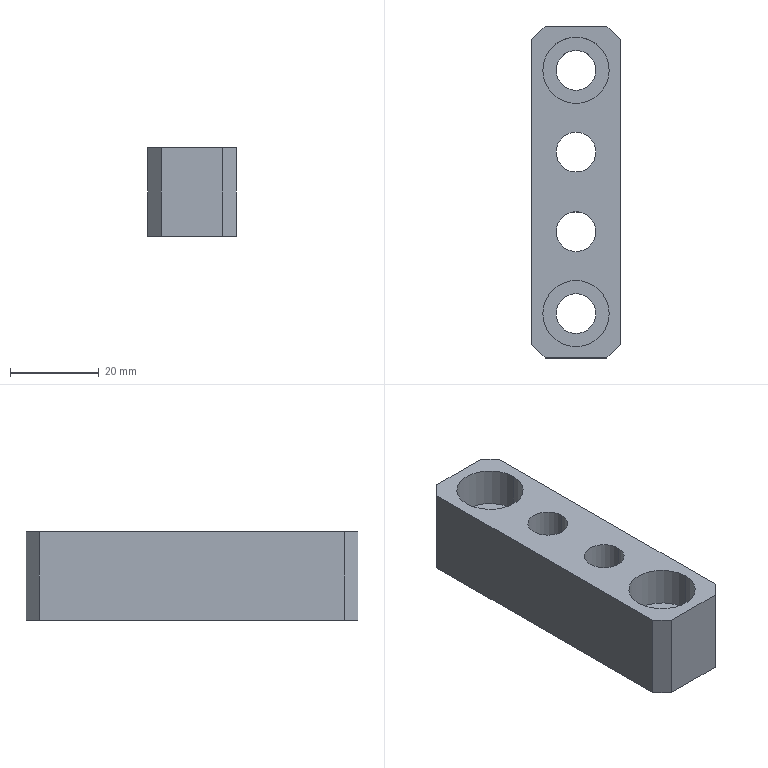Component | SolidWorks | J-TRD899MINI-2213-02BracketVerticalPlate-1 | 1 solid | 30 faces | box 20 x 75 x 20 mm | volume 20479 mm3 | cylinder 16 | plane 14 | commonest cylinder face diameters 15 x8 9 x8 | material 6061
build123d program:
from build123d import *

# Parameters (mm, degrees)
SKETCH1_W                                            = 20
SKETCH1_H                                            = 75
BOSS_EXTRUDE1_DEPTH                                  = 20
HOLE_SIZE_ACCORDING_TO_TYPE_1_OF_HEXAGON_D           = 9
HOLE_SIZE_ACCORDING_TO_TYPE_1_OF_HEXAGON_CBORE_D     = 15
HOLE_SIZE_ACCORDING_TO_TYPE_1_OF_HEXAGON_CBORE_DEPTH = 9
HOLE_SIZE_ACCORDING_TO_TYPE_2_OF_HEXAGON_D           = 9
HOLE_SIZE_ACCORDING_TO_TYPE_2_OF_HEXAGON_CBORE_D     = 15
HOLE_SIZE_ACCORDING_TO_TYPE_2_OF_HEXAGON_CBORE_DEPTH = 9
CHAMFER1_SIZE                                        = 3
CIRPATTERN1_COUNT                                    = 2


with BuildPart() as part:
    # Sketch1 → Boss-Extrude1 (new body)
    with BuildSketch(Plane.XY):
        Rectangle(SKETCH1_W, SKETCH1_H)
    extrude(amount=BOSS_EXTRUDE1_DEPTH)

    # Hole Size_According to_Type 1 of Hexagon (through all)
    with Locations(Plane(origin=(0, 0, 0), x_dir=(-1, 0, 0), z_dir=(0, 0, -1))):
        with Locations((0, 9)):
            hole_size_according_to_type_1_of_hexagon = CounterBoreHole(HOLE_SIZE_ACCORDING_TO_TYPE_1_OF_HEXAGON_D / 2, HOLE_SIZE_ACCORDING_TO_TYPE_1_OF_HEXAGON_CBORE_D / 2, HOLE_SIZE_ACCORDING_TO_TYPE_1_OF_HEXAGON_CBORE_DEPTH)

    # Hole Size_According to_Type 2 of Hexagon (through all)
    with Locations(Plane.XY.offset(20)):
        with Locations((0, 27.5)):
            hole_size_according_to_type_2_of_hexagon = CounterBoreHole(HOLE_SIZE_ACCORDING_TO_TYPE_2_OF_HEXAGON_D / 2, HOLE_SIZE_ACCORDING_TO_TYPE_2_OF_HEXAGON_CBORE_D / 2, HOLE_SIZE_ACCORDING_TO_TYPE_2_OF_HEXAGON_CBORE_DEPTH)

    # Chamfer1
    chamfer1_edges = [part.edges().sort_by_distance(p)[0] for p in [
        (10, -37.5, 10),
        (-10, -37.5, 10),
        (-10, 37.5, 10),
        (10, 37.5, 10),
    ]]
    chamfer(chamfer1_edges, length=CHAMFER1_SIZE)

    # CirPattern1: Hole Size_According to_Type 1 of Hexagon, Hole Size_According to_Type 2 of Hexagon ×2 about axis
    cirpattern1_axis = Axis((0, 0, 0), (0, 0, 1))
    add([hole_size_according_to_type_1_of_hexagon.rotate(cirpattern1_axis, i * 360 / CIRPATTERN1_COUNT) for i in range(1, CIRPATTERN1_COUNT)], mode=Mode.SUBTRACT)
    add([hole_size_according_to_type_2_of_hexagon.rotate(cirpattern1_axis, i * 360 / CIRPATTERN1_COUNT) for i in range(1, CIRPATTERN1_COUNT)], mode=Mode.SUBTRACT)


solid = part.part

# Placed as in the assembly
solid = solid.moved(Location((-6.663, 8.496, 65), (0, 0, 0)))
STEP:
#1=COLOUR_RGB('',0.7922,0.8196,0.9333);
#2=FILL_AREA_STYLE_COLOUR('',#1);
#3=FILL_AREA_STYLE('',(#2));
#4=SURFACE_STYLE_FILL_AREA(#3);
#5=SURFACE_SIDE_STYLE('',(#4));
#6=SURFACE_STYLE_USAGE(.BOTH.,#5);
#7=PRESENTATION_STYLE_ASSIGNMENT((#6));
#8=CARTESIAN_POINT('',(-0.5576,-0.7482,2.992));
#9=VERTEX_POINT('',#8);
#10=CARTESIAN_POINT('',(0.03293,-0.7482,2.992));
#11=VERTEX_POINT('',#10);
#12=CARTESIAN_POINT('',(-0.2623,-0.7482,2.992));
#13=DIRECTION('',(0.,0.,1.));
#14=DIRECTION('',(1.,0.,0.));
#15=AXIS2_PLACEMENT_3D('',#12,#13,#14);
#16=CIRCLE('',#15,0.2953);
#17=EDGE_CURVE('',#9,#11,#16,.T.);
#18=ORIENTED_EDGE('',*,*,#17,.F.);
#19=CARTESIAN_POINT('',(-0.5576,-0.7482,3.346));
#20=VERTEX_POINT('',#19);
#21=CARTESIAN_POINT('',(-0.5576,-0.7482,3.346));
#22=DIRECTION('',(0.,0.,1.));
#23=VECTOR('',#22,39.37);
#24=LINE('',#21,#23);
#25=EDGE_CURVE('',#9,#20,#24,.T.);
#26=ORIENTED_EDGE('',*,*,#25,.T.);
#27=CARTESIAN_POINT('',(0.03293,-0.7482,3.346));
#28=VERTEX_POINT('',#27);
#29=CARTESIAN_POINT('',(-0.2623,-0.7482,3.346));
#30=DIRECTION('',(0.,0.,1.));
#31=DIRECTION('',(1.,0.,0.));
#32=AXIS2_PLACEMENT_3D('',#29,#30,#31);
#33=CIRCLE('',#32,0.2953);
#34=EDGE_CURVE('',#20,#28,#33,.T.);
#35=ORIENTED_EDGE('',*,*,#34,.T.);
#36=CARTESIAN_POINT('',(0.03293,-0.7482,3.346));
#37=DIRECTION('',(0.,0.,1.));
#38=VECTOR('',#37,39.37);
#39=LINE('',#36,#38);
#40=EDGE_CURVE('',#11,#28,#39,.T.);
#41=ORIENTED_EDGE('',*,*,#40,.F.);
#42=EDGE_LOOP('',(#18,#26,#35,#41));
#43=FACE_OUTER_BOUND('',#42,.T.);
#44=CARTESIAN_POINT('',(-0.2623,-0.7482,3.346));
#45=DIRECTION('',(0.,0.,1.));
#46=DIRECTION('',(1.,0.,0.));
#47=AXIS2_PLACEMENT_3D('',#44,#45,#46);
#48=CYLINDRICAL_SURFACE('',#47,0.2953);
#49=ADVANCED_FACE('',(#43),#48,.F.);
#50=CARTESIAN_POINT('',(-0.4395,-0.7482,2.559));
#51=VERTEX_POINT('',#50);
#52=CARTESIAN_POINT('',(-0.08518,-0.7482,2.559));
#53=VERTEX_POINT('',#52);
#54=CARTESIAN_POINT('',(-0.2623,-0.7482,2.559));
#55=DIRECTION('',(0.,0.,1.));
#56=DIRECTION('',(1.,0.,0.));
#57=AXIS2_PLACEMENT_3D('',#54,#55,#56);
#58=CIRCLE('',#57,0.1772);
#59=EDGE_CURVE('',#51,#53,#58,.T.);
#60=ORIENTED_EDGE('',*,*,#59,.F.);
#61=CARTESIAN_POINT('',(-0.4395,-0.7482,2.992));
#62=VERTEX_POINT('',#61);
#63=CARTESIAN_POINT('',(-0.4395,-0.7482,3.346));
#64=DIRECTION('',(0.,0.,1.));
#65=VECTOR('',#64,39.37);
#66=LINE('',#63,#65);
#67=EDGE_CURVE('',#51,#62,#66,.T.);
#68=ORIENTED_EDGE('',*,*,#67,.T.);
#69=CARTESIAN_POINT('',(-0.08518,-0.7482,2.992));
#70=VERTEX_POINT('',#69);
#71=CARTESIAN_POINT('',(-0.2623,-0.7482,2.992));
#72=DIRECTION('',(0.,0.,1.));
#73=DIRECTION('',(1.,0.,0.));
#74=AXIS2_PLACEMENT_3D('',#71,#72,#73);
#75=CIRCLE('',#74,0.1772);
#76=EDGE_CURVE('',#62,#70,#75,.T.);
#77=ORIENTED_EDGE('',*,*,#76,.T.);
#78=CARTESIAN_POINT('',(-0.08518,-0.7482,3.346));
#79=DIRECTION('',(0.,0.,1.));
#80=VECTOR('',#79,39.37);
#81=LINE('',#78,#80);
#82=EDGE_CURVE('',#53,#70,#81,.T.);
#83=ORIENTED_EDGE('',*,*,#82,.F.);
#84=EDGE_LOOP('',(#60,#68,#77,#83));
#85=FACE_OUTER_BOUND('',#84,.T.);
#86=CARTESIAN_POINT('',(-0.2623,-0.7482,3.346));
#87=DIRECTION('',(0.,0.,1.));
#88=DIRECTION('',(1.,0.,0.));
#89=AXIS2_PLACEMENT_3D('',#86,#87,#88);
#90=CYLINDRICAL_SURFACE('',#89,0.1772);
#91=ADVANCED_FACE('',(#85),#90,.F.);
#92=CARTESIAN_POINT('',(0.03293,-0.01984,2.913));
#93=VERTEX_POINT('',#92);
#94=CARTESIAN_POINT('',(-0.5576,-0.01984,2.913));
#95=VERTEX_POINT('',#94);
#96=CARTESIAN_POINT('',(-0.2623,-0.01984,2.913));
#97=DIRECTION('',(0.,0.,-1.));
#98=DIRECTION('',(-1.,0.,0.));
#99=AXIS2_PLACEMENT_3D('',#96,#97,#98);
#100=CIRCLE('',#99,0.2953);
#101=EDGE_CURVE('',#93,#95,#100,.T.);
#102=ORIENTED_EDGE('',*,*,#101,.F.);
#103=CARTESIAN_POINT('',(0.03293,-0.01984,2.559));
#104=VERTEX_POINT('',#103);
#105=CARTESIAN_POINT('',(0.03293,-0.01984,2.559));
#106=DIRECTION('',(0.,0.,-1.));
#107=VECTOR('',#106,39.37);
#108=LINE('',#105,#107);
#109=EDGE_CURVE('',#93,#104,#108,.T.);
#110=ORIENTED_EDGE('',*,*,#109,.T.);
#111=CARTESIAN_POINT('',(-0.5576,-0.01984,2.559));
#112=VERTEX_POINT('',#111);
#113=CARTESIAN_POINT('',(-0.2623,-0.01984,2.559));
#114=DIRECTION('',(0.,0.,-1.));
#115=DIRECTION('',(-1.,0.,0.));
#116=AXIS2_PLACEMENT_3D('',#113,#114,#115);
#117=CIRCLE('',#116,0.2953);
#118=EDGE_CURVE('',#104,#112,#117,.T.);
#119=ORIENTED_EDGE('',*,*,#118,.T.);
#120=CARTESIAN_POINT('',(-0.5576,-0.01984,2.559));
#121=DIRECTION('',(0.,0.,-1.));
#122=VECTOR('',#121,39.37);
#123=LINE('',#120,#122);
#124=EDGE_CURVE('',#95,#112,#123,.T.);
#125=ORIENTED_EDGE('',*,*,#124,.F.);
#126=EDGE_LOOP('',(#102,#110,#119,#125));
#127=FACE_OUTER_BOUND('',#126,.T.);
#128=CARTESIAN_POINT('',(-0.2623,-0.01984,2.559));
#129=DIRECTION('',(0.,0.,-1.));
#130=DIRECTION('',(-1.,0.,0.));
#131=AXIS2_PLACEMENT_3D('',#128,#129,#130);
#132=CYLINDRICAL_SURFACE('',#131,0.2953);
#133=ADVANCED_FACE('',(#127),#132,.F.);
#134=CARTESIAN_POINT('',(-0.08518,-0.01984,3.346));
#135=VERTEX_POINT('',#134);
#136=CARTESIAN_POINT('',(-0.4395,-0.01984,3.346));
#137=VERTEX_POINT('',#136);
#138=CARTESIAN_POINT('',(-0.2623,-0.01984,3.346));
#139=DIRECTION('',(0.,0.,-1.));
#140=DIRECTION('',(-1.,0.,0.));
#141=AXIS2_PLACEMENT_3D('',#138,#139,#140);
#142=CIRCLE('',#141,0.1772);
#143=EDGE_CURVE('',#135,#137,#142,.T.);
#144=ORIENTED_EDGE('',*,*,#143,.F.);
#145=CARTESIAN_POINT('',(-0.08518,-0.01984,2.913));
#146=VERTEX_POINT('',#145);
#147=CARTESIAN_POINT('',(-0.08518,-0.01984,2.559));
#148=DIRECTION('',(0.,0.,-1.));
#149=VECTOR('',#148,39.37);
#150=LINE('',#147,#149);
#151=EDGE_CURVE('',#135,#146,#150,.T.);
#152=ORIENTED_EDGE('',*,*,#151,.T.);
#153=CARTESIAN_POINT('',(-0.4395,-0.01984,2.913));
#154=VERTEX_POINT('',#153);
#155=CARTESIAN_POINT('',(-0.2623,-0.01984,2.913));
#156=DIRECTION('',(0.,0.,-1.));
#157=DIRECTION('',(-1.,0.,0.));
#158=AXIS2_PLACEMENT_3D('',#155,#156,#157);
#159=CIRCLE('',#158,0.1772);
#160=EDGE_CURVE('',#146,#154,#159,.T.);
#161=ORIENTED_EDGE('',*,*,#160,.T.);
#162=CARTESIAN_POINT('',(-0.4395,-0.01984,2.559));
#163=DIRECTION('',(0.,0.,-1.));
#164=VECTOR('',#163,39.37);
#165=LINE('',#162,#164);
#166=EDGE_CURVE('',#137,#154,#165,.T.);
#167=ORIENTED_EDGE('',*,*,#166,.F.);
#168=EDGE_LOOP('',(#144,#152,#161,#167));
#169=FACE_OUTER_BOUND('',#168,.T.);
#170=CARTESIAN_POINT('',(-0.2623,-0.01984,2.559));
#171=DIRECTION('',(0.,0.,-1.));
#172=DIRECTION('',(-1.,0.,0.));
#173=AXIS2_PLACEMENT_3D('',#170,#171,#172);
#174=CYLINDRICAL_SURFACE('',#173,0.1772);
#175=ADVANCED_FACE('',(#169),#174,.F.);
#176=CARTESIAN_POINT('',(-0.5576,1.417,2.992));
#177=VERTEX_POINT('',#176);
#178=CARTESIAN_POINT('',(0.03293,1.417,2.992));
#179=VERTEX_POINT('',#178);
#180=CARTESIAN_POINT('',(-0.2623,1.417,2.992));
#181=DIRECTION('',(0.,0.,1.));
#182=DIRECTION('',(1.,0.,0.));
#183=AXIS2_PLACEMENT_3D('',#180,#181,#182);
#184=CIRCLE('',#183,0.2953);
#185=EDGE_CURVE('',#177,#179,#184,.T.);
#186=ORIENTED_EDGE('',*,*,#185,.F.);
#187=CARTESIAN_POINT('',(-0.5576,1.417,3.346));
#188=VERTEX_POINT('',#187);
#189=CARTESIAN_POINT('',(-0.5576,1.417,3.346));
#190=DIRECTION('',(0.,0.,1.));
#191=VECTOR('',#190,39.37);
#192=LINE('',#189,#191);
#193=EDGE_CURVE('',#177,#188,#192,.T.);
#194=ORIENTED_EDGE('',*,*,#193,.T.);
#195=CARTESIAN_POINT('',(0.03293,1.417,3.346));
#196=VERTEX_POINT('',#195);
#197=CARTESIAN_POINT('',(-0.2623,1.417,3.346));
#198=DIRECTION('',(0.,0.,1.));
#199=DIRECTION('',(1.,0.,0.));
#200=AXIS2_PLACEMENT_3D('',#197,#198,#199);
#201=CIRCLE('',#200,0.2953);
#202=EDGE_CURVE('',#188,#196,#201,.T.);
#203=ORIENTED_EDGE('',*,*,#202,.T.);
#204=CARTESIAN_POINT('',(0.03293,1.417,3.346));
#205=DIRECTION('',(0.,0.,1.));
#206=VECTOR('',#205,39.37);
#207=LINE('',#204,#206);
#208=EDGE_CURVE('',#179,#196,#207,.T.);
#209=ORIENTED_EDGE('',*,*,#208,.F.);
#210=EDGE_LOOP('',(#186,#194,#203,#209));
#211=FACE_OUTER_BOUND('',#210,.T.);
#212=CARTESIAN_POINT('',(-0.2623,1.417,3.346));
#213=DIRECTION('',(0.,0.,1.));
#214=DIRECTION('',(1.,0.,0.));
#215=AXIS2_PLACEMENT_3D('',#212,#213,#214);
#216=CYLINDRICAL_SURFACE('',#215,0.2953);
#217=ADVANCED_FACE('',(#211),#216,.F.);
#218=CARTESIAN_POINT('',(-0.4395,1.417,2.559));
#219=VERTEX_POINT('',#218);
#220=CARTESIAN_POINT('',(-0.08518,1.417,2.559));
#221=VERTEX_POINT('',#220);
#222=CARTESIAN_POINT('',(-0.2623,1.417,2.559));
#223=DIRECTION('',(0.,0.,1.));
#224=DIRECTION('',(1.,0.,0.));
#225=AXIS2_PLACEMENT_3D('',#222,#223,#224);
#226=CIRCLE('',#225,0.1772);
#227=EDGE_CURVE('',#219,#221,#226,.T.);
#228=ORIENTED_EDGE('',*,*,#227,.F.);
#229=CARTESIAN_POINT('',(-0.4395,1.417,2.992));
#230=VERTEX_POINT('',#229);
#231=CARTESIAN_POINT('',(-0.4395,1.417,3.346));
#232=DIRECTION('',(0.,0.,1.));
#233=VECTOR('',#232,39.37);
#234=LINE('',#231,#233);
#235=EDGE_CURVE('',#219,#230,#234,.T.);
#236=ORIENTED_EDGE('',*,*,#235,.T.);
#237=CARTESIAN_POINT('',(-0.08518,1.417,2.992));
#238=VERTEX_POINT('',#237);
#239=CARTESIAN_POINT('',(-0.2623,1.417,2.992));
#240=DIRECTION('',(0.,0.,1.));
#241=DIRECTION('',(1.,0.,0.));
#242=AXIS2_PLACEMENT_3D('',#239,#240,#241);
#243=CIRCLE('',#242,0.1772);
#244=EDGE_CURVE('',#230,#238,#243,.T.);
#245=ORIENTED_EDGE('',*,*,#244,.T.);
#246=CARTESIAN_POINT('',(-0.08518,1.417,3.346));
#247=DIRECTION('',(0.,0.,1.));
#248=VECTOR('',#247,39.37);
#249=LINE('',#246,#248);
#250=EDGE_CURVE('',#221,#238,#249,.T.);
#251=ORIENTED_EDGE('',*,*,#250,.F.);
#252=EDGE_LOOP('',(#228,#236,#245,#251));
#253=FACE_OUTER_BOUND('',#252,.T.);
#254=CARTESIAN_POINT('',(-0.2623,1.417,3.346));
#255=DIRECTION('',(0.,0.,1.));
#256=DIRECTION('',(1.,0.,0.));
#257=AXIS2_PLACEMENT_3D('',#254,#255,#256);
#258=CYLINDRICAL_SURFACE('',#257,0.1772);
#259=ADVANCED_FACE('',(#253),#258,.F.);
#260=CARTESIAN_POINT('',(0.03293,0.6888,2.913));
#261=VERTEX_POINT('',#260);
#262=CARTESIAN_POINT('',(-0.5576,0.6888,2.913));
#263=VERTEX_POINT('',#262);
#264=CARTESIAN_POINT('',(-0.2623,0.6888,2.913));
#265=DIRECTION('',(0.,0.,-1.));
#266=DIRECTION('',(-1.,0.,0.));
#267=AXIS2_PLACEMENT_3D('',#264,#265,#266);
#268=CIRCLE('',#267,0.2953);
#269=EDGE_CURVE('',#261,#263,#268,.T.);
#270=ORIENTED_EDGE('',*,*,#269,.F.);
#271=CARTESIAN_POINT('',(0.03293,0.6888,2.559));
#272=VERTEX_POINT('',#271);
#273=CARTESIAN_POINT('',(0.03293,0.6888,2.559));
#274=DIRECTION('',(0.,0.,-1.));
#275=VECTOR('',#274,39.37);
#276=LINE('',#273,#275);
#277=EDGE_CURVE('',#261,#272,#276,.T.);
#278=ORIENTED_EDGE('',*,*,#277,.T.);
#279=CARTESIAN_POINT('',(-0.5576,0.6888,2.559));
#280=VERTEX_POINT('',#279);
#281=CARTESIAN_POINT('',(-0.2623,0.6888,2.559));
#282=DIRECTION('',(0.,0.,-1.));
#283=DIRECTION('',(-1.,0.,0.));
#284=AXIS2_PLACEMENT_3D('',#281,#282,#283);
#285=CIRCLE('',#284,0.2953);
#286=EDGE_CURVE('',#272,#280,#285,.T.);
#287=ORIENTED_EDGE('',*,*,#286,.T.);
#288=CARTESIAN_POINT('',(-0.5576,0.6888,2.559));
#289=DIRECTION('',(0.,0.,-1.));
#290=VECTOR('',#289,39.37);
#291=LINE('',#288,#290);
#292=EDGE_CURVE('',#263,#280,#291,.T.);
#293=ORIENTED_EDGE('',*,*,#292,.F.);
#294=EDGE_LOOP('',(#270,#278,#287,#293));
#295=FACE_OUTER_BOUND('',#294,.T.);
#296=CARTESIAN_POINT('',(-0.2623,0.6888,2.559));
#297=DIRECTION('',(0.,0.,-1.));
#298=DIRECTION('',(-1.,0.,0.));
#299=AXIS2_PLACEMENT_3D('',#296,#297,#298);
#300=CYLINDRICAL_SURFACE('',#299,0.2953);
#301=ADVANCED_FACE('',(#295),#300,.F.);
#302=CARTESIAN_POINT('',(-0.08518,0.6888,3.346));
#303=VERTEX_POINT('',#302);
#304=CARTESIAN_POINT('',(-0.4395,0.6888,3.346));
#305=VERTEX_POINT('',#304);
#306=CARTESIAN_POINT('',(-0.2623,0.6888,3.346));
#307=DIRECTION('',(0.,0.,-1.));
#308=DIRECTION('',(-1.,0.,0.));
#309=AXIS2_PLACEMENT_3D('',#306,#307,#308);
#310=CIRCLE('',#309,0.1772);
#311=EDGE_CURVE('',#303,#305,#310,.T.);
#312=ORIENTED_EDGE('',*,*,#311,.F.);
#313=CARTESIAN_POINT('',(-0.08518,0.6888,2.913));
#314=VERTEX_POINT('',#313);
#315=CARTESIAN_POINT('',(-0.08518,0.6888,2.559));
#316=DIRECTION('',(0.,0.,-1.));
#317=VECTOR('',#316,39.37);
#318=LINE('',#315,#317);
#319=EDGE_CURVE('',#303,#314,#318,.T.);
#320=ORIENTED_EDGE('',*,*,#319,.T.);
#321=CARTESIAN_POINT('',(-0.4395,0.6888,2.913));
#322=VERTEX_POINT('',#321);
#323=CARTESIAN_POINT('',(-0.2623,0.6888,2.913));
#324=DIRECTION('',(0.,0.,-1.));
#325=DIRECTION('',(-1.,0.,0.));
#326=AXIS2_PLACEMENT_3D('',#323,#324,#325);
#327=CIRCLE('',#326,0.1772);
#328=EDGE_CURVE('',#314,#322,#327,.T.);
#329=ORIENTED_EDGE('',*,*,#328,.T.);
#330=CARTESIAN_POINT('',(-0.4395,0.6888,2.559));
#331=DIRECTION('',(0.,0.,-1.));
#332=VECTOR('',#331,39.37);
#333=LINE('',#330,#332);
#334=EDGE_CURVE('',#305,#322,#333,.T.);
#335=ORIENTED_EDGE('',*,*,#334,.F.);
#336=EDGE_LOOP('',(#312,#320,#329,#335));
#337=FACE_OUTER_BOUND('',#336,.T.);
#338=CARTESIAN_POINT('',(-0.2623,0.6888,2.559));
#339=DIRECTION('',(0.,0.,-1.));
#340=DIRECTION('',(-1.,0.,0.));
#341=AXIS2_PLACEMENT_3D('',#338,#339,#340);
#342=CYLINDRICAL_SURFACE('',#341,0.1772);
#343=ADVANCED_FACE('',(#337),#342,.F.);
#344=CARTESIAN_POINT('',(0.1314,-1.024,3.346));
#345=VERTEX_POINT('',#344);
#346=CARTESIAN_POINT('',(0.1314,1.693,3.346));
#347=VERTEX_POINT('',#346);
#348=CARTESIAN_POINT('',(0.1314,-1.142,3.346));
#349=DIRECTION('',(0.,1.,0.));
#350=VECTOR('',#349,39.37);
#351=LINE('',#348,#350);
#352=EDGE_CURVE('',#345,#347,#351,.T.);
#353=ORIENTED_EDGE('',*,*,#352,.F.);
#354=CARTESIAN_POINT('',(0.1314,-1.024,2.559));
#355=VERTEX_POINT('',#354);
#356=CARTESIAN_POINT('',(0.1314,-1.024,3.346));
#357=DIRECTION('',(0.,0.,-1.));
#358=VECTOR('',#357,39.37);
#359=LINE('',#356,#358);
#360=EDGE_CURVE('',#345,#355,#359,.T.);
#361=ORIENTED_EDGE('',*,*,#360,.T.);
#362=CARTESIAN_POINT('',(0.1314,1.693,2.559));
#363=VERTEX_POINT('',#362);
#364=CARTESIAN_POINT('',(0.1314,-1.142,2.559));
#365=DIRECTION('',(0.,1.,0.));
#366=VECTOR('',#365,39.37);
#367=LINE('',#364,#366);
#368=EDGE_CURVE('',#355,#363,#367,.T.);
#369=ORIENTED_EDGE('',*,*,#368,.T.);
#370=CARTESIAN_POINT('',(0.1314,1.693,3.346));
#371=DIRECTION('',(0.,0.,1.));
#372=VECTOR('',#371,39.37);
#373=LINE('',#370,#372);
#374=EDGE_CURVE('',#363,#347,#373,.T.);
#375=ORIENTED_EDGE('',*,*,#374,.T.);
#376=EDGE_LOOP('',(#353,#361,#369,#375));
#377=FACE_OUTER_BOUND('',#376,.T.);
#378=CARTESIAN_POINT('',(0.1314,-1.142,3.346));
#379=DIRECTION('',(-1.,0.,0.));
#380=DIRECTION('',(0.,0.,1.));
#381=AXIS2_PLACEMENT_3D('',#378,#379,#380);
#382=PLANE('',#381);
#383=ADVANCED_FACE('',(#377),#382,.F.);
#384=CARTESIAN_POINT('',(0.01325,1.811,3.346));
#385=VERTEX_POINT('',#384);
#386=CARTESIAN_POINT('',(-0.5379,1.811,3.346));
#387=VERTEX_POINT('',#386);
#388=CARTESIAN_POINT('',(-0.656,1.811,3.346));
#389=DIRECTION('',(-1.,0.,0.));
#390=VECTOR('',#389,39.37);
#391=LINE('',#388,#390);
#392=EDGE_CURVE('',#385,#387,#391,.T.);
#393=ORIENTED_EDGE('',*,*,#392,.F.);
#394=CARTESIAN_POINT('',(0.01325,1.811,2.559));
#395=VERTEX_POINT('',#394);
#396=CARTESIAN_POINT('',(0.01325,1.811,3.346));
#397=DIRECTION('',(0.,0.,-1.));
#398=VECTOR('',#397,39.37);
#399=LINE('',#396,#398);
#400=EDGE_CURVE('',#385,#395,#399,.T.);
#401=ORIENTED_EDGE('',*,*,#400,.T.);
#402=CARTESIAN_POINT('',(-0.5379,1.811,2.559));
#403=VERTEX_POINT('',#402);
#404=CARTESIAN_POINT('',(-0.656,1.811,2.559));
#405=DIRECTION('',(-1.,0.,0.));
#406=VECTOR('',#405,39.37);
#407=LINE('',#404,#406);
#408=EDGE_CURVE('',#395,#403,#407,.T.);
#409=ORIENTED_EDGE('',*,*,#408,.T.);
#410=CARTESIAN_POINT('',(-0.5379,1.811,3.346));
#411=DIRECTION('',(0.,0.,1.));
#412=VECTOR('',#411,39.37);
#413=LINE('',#410,#412);
#414=EDGE_CURVE('',#403,#387,#413,.T.);
#415=ORIENTED_EDGE('',*,*,#414,.T.);
#416=EDGE_LOOP('',(#393,#401,#409,#415));
#417=FACE_OUTER_BOUND('',#416,.T.);
#418=CARTESIAN_POINT('',(-0.656,1.811,3.346));
#419=DIRECTION('',(0.,-1.,0.));
#420=DIRECTION('',(0.,0.,-1.));
#421=AXIS2_PLACEMENT_3D('',#418,#419,#420);
#422=PLANE('',#421);
#423=ADVANCED_FACE('',(#417),#422,.F.);
#424=CARTESIAN_POINT('',(-0.656,1.693,2.559));
#425=VERTEX_POINT('',#424);
#426=CARTESIAN_POINT('',(-0.656,-1.024,2.559));
#427=VERTEX_POINT('',#426);
#428=CARTESIAN_POINT('',(-0.656,-1.142,2.559));
#429=DIRECTION('',(0.,-1.,0.));
#430=VECTOR('',#429,39.37);
#431=LINE('',#428,#430);
#432=EDGE_CURVE('',#425,#427,#431,.T.);
#433=ORIENTED_EDGE('',*,*,#432,.T.);
#434=CARTESIAN_POINT('',(-0.656,-1.024,3.346));
#435=VERTEX_POINT('',#434);
#436=CARTESIAN_POINT('',(-0.656,-1.024,3.346));
#437=DIRECTION('',(0.,0.,1.));
#438=VECTOR('',#437,39.37);
#439=LINE('',#436,#438);
#440=EDGE_CURVE('',#427,#435,#439,.T.);
#441=ORIENTED_EDGE('',*,*,#440,.T.);
#442=CARTESIAN_POINT('',(-0.656,1.693,3.346));
#443=VERTEX_POINT('',#442);
#444=CARTESIAN_POINT('',(-0.656,-1.142,3.346));
#445=DIRECTION('',(0.,-1.,0.));
#446=VECTOR('',#445,39.37);
#447=LINE('',#444,#446);
#448=EDGE_CURVE('',#443,#435,#447,.T.);
#449=ORIENTED_EDGE('',*,*,#448,.F.);
#450=CARTESIAN_POINT('',(-0.656,1.693,3.346));
#451=DIRECTION('',(0.,0.,-1.));
#452=VECTOR('',#451,39.37);
#453=LINE('',#450,#452);
#454=EDGE_CURVE('',#443,#425,#453,.T.);
#455=ORIENTED_EDGE('',*,*,#454,.T.);
#456=EDGE_LOOP('',(#433,#441,#449,#455));
#457=FACE_OUTER_BOUND('',#456,.T.);
#458=CARTESIAN_POINT('',(-0.656,-1.142,3.346));
#459=DIRECTION('',(1.,0.,0.));
#460=DIRECTION('',(0.,0.,-1.));
#461=AXIS2_PLACEMENT_3D('',#458,#459,#460);
#462=PLANE('',#461);
#463=ADVANCED_FACE('',(#457),#462,.F.);
#464=CARTESIAN_POINT('',(-0.5379,-1.142,3.346));
#465=VERTEX_POINT('',#464);
#466=CARTESIAN_POINT('',(0.01325,-1.142,3.346));
#467=VERTEX_POINT('',#466);
#468=CARTESIAN_POINT('',(-0.656,-1.142,3.346));
#469=DIRECTION('',(1.,0.,0.));
#470=VECTOR('',#469,39.37);
#471=LINE('',#468,#470);
#472=EDGE_CURVE('',#465,#467,#471,.T.);
#473=ORIENTED_EDGE('',*,*,#472,.F.);
#474=CARTESIAN_POINT('',(-0.5379,-1.142,2.559));
#475=VERTEX_POINT('',#474);
#476=CARTESIAN_POINT('',(-0.5379,-1.142,3.346));
#477=DIRECTION('',(0.,0.,-1.));
#478=VECTOR('',#477,39.37);
#479=LINE('',#476,#478);
#480=EDGE_CURVE('',#465,#475,#479,.T.);
#481=ORIENTED_EDGE('',*,*,#480,.T.);
#482=CARTESIAN_POINT('',(0.01325,-1.142,2.559));
#483=VERTEX_POINT('',#482);
#484=CARTESIAN_POINT('',(-0.656,-1.142,2.559));
#485=DIRECTION('',(1.,0.,0.));
#486=VECTOR('',#485,39.37);
#487=LINE('',#484,#486);
#488=EDGE_CURVE('',#475,#483,#487,.T.);
#489=ORIENTED_EDGE('',*,*,#488,.T.);
#490=CARTESIAN_POINT('',(0.01325,-1.142,3.346));
#491=DIRECTION('',(0.,0.,1.));
#492=VECTOR('',#491,39.37);
#493=LINE('',#490,#492);
#494=EDGE_CURVE('',#483,#467,#493,.T.);
#495=ORIENTED_EDGE('',*,*,#494,.T.);
#496=EDGE_LOOP('',(#473,#481,#489,#495));
#497=FACE_OUTER_BOUND('',#496,.T.);
#498=CARTESIAN_POINT('',(-0.656,-1.142,3.346));
#499=DIRECTION('',(0.,1.,0.));
#500=DIRECTION('',(0.,0.,1.));
#501=AXIS2_PLACEMENT_3D('',#498,#499,#500);
#502=PLANE('',#501);
#503=ADVANCED_FACE('',(#497),#502,.F.);
#504=CARTESIAN_POINT('',(-0.2623,-0.7482,3.346));
#505=DIRECTION('',(0.,0.,1.));
#506=DIRECTION('',(1.,0.,0.));
#507=AXIS2_PLACEMENT_3D('',#504,#505,#506);
#508=CIRCLE('',#507,0.2953);
#509=EDGE_CURVE('',#28,#20,#508,.T.);
#510=ORIENTED_EDGE('',*,*,#509,.F.);
#511=ORIENTED_EDGE('',*,*,#34,.F.);
#512=EDGE_LOOP('',(#510,#511));
#513=FACE_BOUND('',#512,.T.);
#514=CARTESIAN_POINT('',(-0.2623,-0.01984,3.346));
#515=DIRECTION('',(0.,0.,-1.));
#516=DIRECTION('',(-1.,0.,0.));
#517=AXIS2_PLACEMENT_3D('',#514,#515,#516);
#518=CIRCLE('',#517,0.1772);
#519=EDGE_CURVE('',#137,#135,#518,.T.);
#520=ORIENTED_EDGE('',*,*,#519,.T.);
#521=ORIENTED_EDGE('',*,*,#143,.T.);
#522=EDGE_LOOP('',(#520,#521));
#523=FACE_BOUND('',#522,.T.);
#524=CARTESIAN_POINT('',(-0.2623,1.417,3.346));
#525=DIRECTION('',(0.,0.,1.));
#526=DIRECTION('',(1.,0.,0.));
#527=AXIS2_PLACEMENT_3D('',#524,#525,#526);
#528=CIRCLE('',#527,0.2953);
#529=EDGE_CURVE('',#196,#188,#528,.T.);
#530=ORIENTED_EDGE('',*,*,#529,.F.);
#531=ORIENTED_EDGE('',*,*,#202,.F.);
#532=EDGE_LOOP('',(#530,#531));
#533=FACE_BOUND('',#532,.T.);
#534=CARTESIAN_POINT('',(-0.2623,0.6888,3.346));
#535=DIRECTION('',(0.,0.,-1.));
#536=DIRECTION('',(-1.,0.,0.));
#537=AXIS2_PLACEMENT_3D('',#534,#535,#536);
#538=CIRCLE('',#537,0.1772);
#539=EDGE_CURVE('',#305,#303,#538,.T.);
#540=ORIENTED_EDGE('',*,*,#539,.T.);
#541=ORIENTED_EDGE('',*,*,#311,.T.);
#542=EDGE_LOOP('',(#540,#541));
#543=FACE_BOUND('',#542,.T.);
#544=ORIENTED_EDGE('',*,*,#448,.T.);
#545=CARTESIAN_POINT('',(-0.5379,-1.142,3.346));
#546=DIRECTION('',(0.7071,-0.7071,0.));
#547=VECTOR('',#546,39.37);
#548=LINE('',#545,#547);
#549=EDGE_CURVE('',#435,#465,#548,.T.);
#550=ORIENTED_EDGE('',*,*,#549,.T.);
#551=ORIENTED_EDGE('',*,*,#472,.T.);
#552=CARTESIAN_POINT('',(0.1314,-1.024,3.346));
#553=DIRECTION('',(0.7071,0.7071,0.));
#554=VECTOR('',#553,39.37);
#555=LINE('',#552,#554);
#556=EDGE_CURVE('',#467,#345,#555,.T.);
#557=ORIENTED_EDGE('',*,*,#556,.T.);
#558=ORIENTED_EDGE('',*,*,#352,.T.);
#559=CARTESIAN_POINT('',(0.01325,1.811,3.346));
#560=DIRECTION('',(-0.7071,0.7071,0.));
#561=VECTOR('',#560,39.37);
#562=LINE('',#559,#561);
#563=EDGE_CURVE('',#347,#385,#562,.T.);
#564=ORIENTED_EDGE('',*,*,#563,.T.);
#565=ORIENTED_EDGE('',*,*,#392,.T.);
#566=CARTESIAN_POINT('',(-0.656,1.693,3.346));
#567=DIRECTION('',(-0.7071,-0.7071,0.));
#568=VECTOR('',#567,39.37);
#569=LINE('',#566,#568);
#570=EDGE_CURVE('',#387,#443,#569,.T.);
#571=ORIENTED_EDGE('',*,*,#570,.T.);
#572=EDGE_LOOP('',(#544,#550,#551,#557,#558,#564,#565,#571));
#573=FACE_OUTER_BOUND('',#572,.T.);
#574=CARTESIAN_POINT('',(-0.2623,0.3345,3.346));
#575=DIRECTION('',(0.,0.,-1.));
#576=DIRECTION('',(-1.,0.,0.));
#577=AXIS2_PLACEMENT_3D('',#574,#575,#576);
#578=PLANE('',#577);
#579=ADVANCED_FACE('',(#513,#523,#533,#543,#573),#578,.F.);
#580=CARTESIAN_POINT('',(-0.2623,-0.7482,2.559));
#581=DIRECTION('',(0.,0.,1.));
#582=DIRECTION('',(1.,0.,0.));
#583=AXIS2_PLACEMENT_3D('',#580,#581,#582);
#584=CIRCLE('',#583,0.1772);
#585=EDGE_CURVE('',#53,#51,#584,.T.);
#586=ORIENTED_EDGE('',*,*,#585,.T.);
#587=ORIENTED_EDGE('',*,*,#59,.T.);
#588=EDGE_LOOP('',(#586,#587));
#589=FACE_BOUND('',#588,.T.);
#590=CARTESIAN_POINT('',(-0.2623,-0.01984,2.559));
#591=DIRECTION('',(0.,0.,-1.));
#592=DIRECTION('',(-1.,0.,0.));
#593=AXIS2_PLACEMENT_3D('',#590,#591,#592);
#594=CIRCLE('',#593,0.2953);
#595=EDGE_CURVE('',#112,#104,#594,.T.);
#596=ORIENTED_EDGE('',*,*,#595,.F.);
#597=ORIENTED_EDGE('',*,*,#118,.F.);
#598=EDGE_LOOP('',(#596,#597));
#599=FACE_BOUND('',#598,.T.);
#600=CARTESIAN_POINT('',(-0.2623,1.417,2.559));
#601=DIRECTION('',(0.,0.,1.));
#602=DIRECTION('',(1.,0.,0.));
#603=AXIS2_PLACEMENT_3D('',#600,#601,#602);
#604=CIRCLE('',#603,0.1772);
#605=EDGE_CURVE('',#221,#219,#604,.T.);
#606=ORIENTED_EDGE('',*,*,#605,.T.);
#607=ORIENTED_EDGE('',*,*,#227,.T.);
#608=EDGE_LOOP('',(#606,#607));
#609=FACE_BOUND('',#608,.T.);
#610=CARTESIAN_POINT('',(-0.2623,0.6888,2.559));
#611=DIRECTION('',(0.,0.,-1.));
#612=DIRECTION('',(-1.,0.,0.));
#613=AXIS2_PLACEMENT_3D('',#610,#611,#612);
#614=CIRCLE('',#613,0.2953);
#615=EDGE_CURVE('',#280,#272,#614,.T.);
#616=ORIENTED_EDGE('',*,*,#615,.F.);
#617=ORIENTED_EDGE('',*,*,#286,.F.);
#618=EDGE_LOOP('',(#616,#617));
#619=FACE_BOUND('',#618,.T.);
#620=ORIENTED_EDGE('',*,*,#488,.F.);
#621=CARTESIAN_POINT('',(-1.138,-0.5415,2.559));
#622=DIRECTION('',(-0.7071,0.7071,0.));
#623=VECTOR('',#622,39.37);
#624=LINE('',#621,#623);
#625=EDGE_CURVE('',#475,#427,#624,.T.);
#626=ORIENTED_EDGE('',*,*,#625,.T.);
#627=ORIENTED_EDGE('',*,*,#432,.F.);
#628=CARTESIAN_POINT('',(-1.138,1.21,2.559));
#629=DIRECTION('',(0.7071,0.7071,0.));
#630=VECTOR('',#629,39.37);
#631=LINE('',#628,#630);
#632=EDGE_CURVE('',#425,#403,#631,.T.);
#633=ORIENTED_EDGE('',*,*,#632,.T.);
#634=ORIENTED_EDGE('',*,*,#408,.F.);
#635=CARTESIAN_POINT('',(0.6136,1.21,2.559));
#636=DIRECTION('',(0.7071,-0.7071,0.));
#637=VECTOR('',#636,39.37);
#638=LINE('',#635,#637);
#639=EDGE_CURVE('',#395,#363,#638,.T.);
#640=ORIENTED_EDGE('',*,*,#639,.T.);
#641=ORIENTED_EDGE('',*,*,#368,.F.);
#642=CARTESIAN_POINT('',(0.6136,-0.5415,2.559));
#643=DIRECTION('',(-0.7071,-0.7071,0.));
#644=VECTOR('',#643,39.37);
#645=LINE('',#642,#644);
#646=EDGE_CURVE('',#355,#483,#645,.T.);
#647=ORIENTED_EDGE('',*,*,#646,.T.);
#648=EDGE_LOOP('',(#620,#626,#627,#633,#634,#640,#641,#647));
#649=FACE_OUTER_BOUND('',#648,.T.);
#650=CARTESIAN_POINT('',(-0.2623,0.3345,2.559));
#651=DIRECTION('',(0.,0.,-1.));
#652=DIRECTION('',(-1.,0.,0.));
#653=AXIS2_PLACEMENT_3D('',#650,#651,#652);
#654=PLANE('',#653);
#655=ADVANCED_FACE('',(#589,#599,#609,#619,#649),#654,.T.);
#656=ORIENTED_EDGE('',*,*,#319,.F.);
#657=ORIENTED_EDGE('',*,*,#539,.F.);
#658=ORIENTED_EDGE('',*,*,#334,.T.);
#659=CARTESIAN_POINT('',(-0.2623,0.6888,2.913));
#660=DIRECTION('',(0.,0.,-1.));
#661=DIRECTION('',(-1.,0.,0.));
#662=AXIS2_PLACEMENT_3D('',#659,#660,#661);
#663=CIRCLE('',#662,0.1772);
#664=EDGE_CURVE('',#322,#314,#663,.T.);
#665=ORIENTED_EDGE('',*,*,#664,.T.);
#666=EDGE_LOOP('',(#656,#657,#658,#665));
#667=FACE_OUTER_BOUND('',#666,.T.);
#668=CARTESIAN_POINT('',(-0.2623,0.6888,2.559));
#669=DIRECTION('',(0.,0.,-1.));
#670=DIRECTION('',(-1.,0.,0.));
#671=AXIS2_PLACEMENT_3D('',#668,#669,#670);
#672=CYLINDRICAL_SURFACE('',#671,0.1772);
#673=ADVANCED_FACE('',(#667),#672,.F.);
#674=ORIENTED_EDGE('',*,*,#664,.F.);
#675=ORIENTED_EDGE('',*,*,#328,.F.);
#676=EDGE_LOOP('',(#674,#675));
#677=FACE_BOUND('',#676,.T.);
#678=CARTESIAN_POINT('',(-0.2623,0.6888,2.913));
#679=DIRECTION('',(0.,0.,-1.));
#680=DIRECTION('',(-1.,0.,0.));
#681=AXIS2_PLACEMENT_3D('',#678,#679,#680);
#682=CIRCLE('',#681,0.2953);
#683=EDGE_CURVE('',#263,#261,#682,.T.);
#684=ORIENTED_EDGE('',*,*,#683,.T.);
#685=ORIENTED_EDGE('',*,*,#269,.T.);
#686=EDGE_LOOP('',(#684,#685));
#687=FACE_OUTER_BOUND('',#686,.T.);
#688=CARTESIAN_POINT('',(-0.08518,0.6888,2.913));
#689=DIRECTION('',(0.,0.,1.));
#690=DIRECTION('',(1.,0.,0.));
#691=AXIS2_PLACEMENT_3D('',#688,#689,#690);
#692=PLANE('',#691);
#693=ADVANCED_FACE('',(#677,#687),#692,.F.);
#694=ORIENTED_EDGE('',*,*,#277,.F.);
#695=ORIENTED_EDGE('',*,*,#683,.F.);
#696=ORIENTED_EDGE('',*,*,#292,.T.);
#697=ORIENTED_EDGE('',*,*,#615,.T.);
#698=EDGE_LOOP('',(#694,#695,#696,#697));
#699=FACE_OUTER_BOUND('',#698,.T.);
#700=CARTESIAN_POINT('',(-0.2623,0.6888,2.559));
#701=DIRECTION('',(0.,0.,-1.));
#702=DIRECTION('',(-1.,0.,0.));
#703=AXIS2_PLACEMENT_3D('',#700,#701,#702);
#704=CYLINDRICAL_SURFACE('',#703,0.2953);
#705=ADVANCED_FACE('',(#699),#704,.F.);
#706=ORIENTED_EDGE('',*,*,#235,.F.);
#707=ORIENTED_EDGE('',*,*,#605,.F.);
#708=ORIENTED_EDGE('',*,*,#250,.T.);
#709=CARTESIAN_POINT('',(-0.2623,1.417,2.992));
#710=DIRECTION('',(0.,0.,1.));
#711=DIRECTION('',(1.,0.,0.));
#712=AXIS2_PLACEMENT_3D('',#709,#710,#711);
#713=CIRCLE('',#712,0.1772);
#714=EDGE_CURVE('',#238,#230,#713,.T.);
#715=ORIENTED_EDGE('',*,*,#714,.T.);
#716=EDGE_LOOP('',(#706,#707,#708,#715));
#717=FACE_OUTER_BOUND('',#716,.T.);
#718=CARTESIAN_POINT('',(-0.2623,1.417,3.346));
#719=DIRECTION('',(0.,0.,1.));
#720=DIRECTION('',(1.,0.,0.));
#721=AXIS2_PLACEMENT_3D('',#718,#719,#720);
#722=CYLINDRICAL_SURFACE('',#721,0.1772);
#723=ADVANCED_FACE('',(#717),#722,.F.);
#724=ORIENTED_EDGE('',*,*,#714,.F.);
#725=ORIENTED_EDGE('',*,*,#244,.F.);
#726=EDGE_LOOP('',(#724,#725));
#727=FACE_BOUND('',#726,.T.);
#728=CARTESIAN_POINT('',(-0.2623,1.417,2.992));
#729=DIRECTION('',(0.,0.,1.));
#730=DIRECTION('',(1.,0.,0.));
#731=AXIS2_PLACEMENT_3D('',#728,#729,#730);
#732=CIRCLE('',#731,0.2953);
#733=EDGE_CURVE('',#179,#177,#732,.T.);
#734=ORIENTED_EDGE('',*,*,#733,.T.);
#735=ORIENTED_EDGE('',*,*,#185,.T.);
#736=EDGE_LOOP('',(#734,#735));
#737=FACE_OUTER_BOUND('',#736,.T.);
#738=CARTESIAN_POINT('',(-0.08518,1.417,2.992));
#739=DIRECTION('',(0.,0.,-1.));
#740=DIRECTION('',(-1.,0.,0.));
#741=AXIS2_PLACEMENT_3D('',#738,#739,#740);
#742=PLANE('',#741);
#743=ADVANCED_FACE('',(#727,#737),#742,.F.);
#744=ORIENTED_EDGE('',*,*,#193,.F.);
#745=ORIENTED_EDGE('',*,*,#733,.F.);
#746=ORIENTED_EDGE('',*,*,#208,.T.);
#747=ORIENTED_EDGE('',*,*,#529,.T.);
#748=EDGE_LOOP('',(#744,#745,#746,#747));
#749=FACE_OUTER_BOUND('',#748,.T.);
#750=CARTESIAN_POINT('',(-0.2623,1.417,3.346));
#751=DIRECTION('',(0.,0.,1.));
#752=DIRECTION('',(1.,0.,0.));
#753=AXIS2_PLACEMENT_3D('',#750,#751,#752);
#754=CYLINDRICAL_SURFACE('',#753,0.2953);
#755=ADVANCED_FACE('',(#749),#754,.F.);
#756=ORIENTED_EDGE('',*,*,#549,.F.);
#757=ORIENTED_EDGE('',*,*,#440,.F.);
#758=ORIENTED_EDGE('',*,*,#625,.F.);
#759=ORIENTED_EDGE('',*,*,#480,.F.);
#760=EDGE_LOOP('',(#756,#757,#758,#759));
#761=FACE_OUTER_BOUND('',#760,.T.);
#762=CARTESIAN_POINT('',(-0.5379,-1.142,3.346));
#763=DIRECTION('',(0.7071,0.7071,0.));
#764=DIRECTION('',(0.,0.,-1.));
#765=AXIS2_PLACEMENT_3D('',#762,#763,#764);
#766=PLANE('',#765);
#767=ADVANCED_FACE('',(#761),#766,.F.);
#768=ORIENTED_EDGE('',*,*,#556,.F.);
#769=ORIENTED_EDGE('',*,*,#494,.F.);
#770=ORIENTED_EDGE('',*,*,#646,.F.);
#771=ORIENTED_EDGE('',*,*,#360,.F.);
#772=EDGE_LOOP('',(#768,#769,#770,#771));
#773=FACE_OUTER_BOUND('',#772,.T.);
#774=CARTESIAN_POINT('',(0.1314,-1.024,3.346));
#775=DIRECTION('',(-0.7071,0.7071,0.));
#776=DIRECTION('',(0.,0.,-1.));
#777=AXIS2_PLACEMENT_3D('',#774,#775,#776);
#778=PLANE('',#777);
#779=ADVANCED_FACE('',(#773),#778,.F.);
#780=ORIENTED_EDGE('',*,*,#563,.F.);
#781=ORIENTED_EDGE('',*,*,#374,.F.);
#782=ORIENTED_EDGE('',*,*,#639,.F.);
#783=ORIENTED_EDGE('',*,*,#400,.F.);
#784=EDGE_LOOP('',(#780,#781,#782,#783));
#785=FACE_OUTER_BOUND('',#784,.T.);
#786=CARTESIAN_POINT('',(0.01325,1.811,3.346));
#787=DIRECTION('',(-0.7071,-0.7071,0.));
#788=DIRECTION('',(0.,0.,-1.));
#789=AXIS2_PLACEMENT_3D('',#786,#787,#788);
#790=PLANE('',#789);
#791=ADVANCED_FACE('',(#785),#790,.F.);
#792=ORIENTED_EDGE('',*,*,#570,.F.);
#793=ORIENTED_EDGE('',*,*,#414,.F.);
#794=ORIENTED_EDGE('',*,*,#632,.F.);
#795=ORIENTED_EDGE('',*,*,#454,.F.);
#796=EDGE_LOOP('',(#792,#793,#794,#795));
#797=FACE_OUTER_BOUND('',#796,.T.);
#798=CARTESIAN_POINT('',(-0.656,1.693,3.346));
#799=DIRECTION('',(0.7071,-0.7071,0.));
#800=DIRECTION('',(0.,0.,-1.));
#801=AXIS2_PLACEMENT_3D('',#798,#799,#800);
#802=PLANE('',#801);
#803=ADVANCED_FACE('',(#797),#802,.F.);
#804=ORIENTED_EDGE('',*,*,#151,.F.);
#805=ORIENTED_EDGE('',*,*,#519,.F.);
#806=ORIENTED_EDGE('',*,*,#166,.T.);
#807=CARTESIAN_POINT('',(-0.2623,-0.01984,2.913));
#808=DIRECTION('',(0.,0.,-1.));
#809=DIRECTION('',(-1.,0.,0.));
#810=AXIS2_PLACEMENT_3D('',#807,#808,#809);
#811=CIRCLE('',#810,0.1772);
#812=EDGE_CURVE('',#154,#146,#811,.T.);
#813=ORIENTED_EDGE('',*,*,#812,.T.);
#814=EDGE_LOOP('',(#804,#805,#806,#813));
#815=FACE_OUTER_BOUND('',#814,.T.);
#816=CARTESIAN_POINT('',(-0.2623,-0.01984,2.559));
#817=DIRECTION('',(0.,0.,-1.));
#818=DIRECTION('',(-1.,0.,0.));
#819=AXIS2_PLACEMENT_3D('',#816,#817,#818);
#820=CYLINDRICAL_SURFACE('',#819,0.1772);
#821=ADVANCED_FACE('',(#815),#820,.F.);
#822=ORIENTED_EDGE('',*,*,#812,.F.);
#823=ORIENTED_EDGE('',*,*,#160,.F.);
#824=EDGE_LOOP('',(#822,#823));
#825=FACE_BOUND('',#824,.T.);
#826=CARTESIAN_POINT('',(-0.2623,-0.01984,2.913));
#827=DIRECTION('',(0.,0.,-1.));
#828=DIRECTION('',(-1.,0.,0.));
#829=AXIS2_PLACEMENT_3D('',#826,#827,#828);
#830=CIRCLE('',#829,0.2953);
#831=EDGE_CURVE('',#95,#93,#830,.T.);
#832=ORIENTED_EDGE('',*,*,#831,.T.);
#833=ORIENTED_EDGE('',*,*,#101,.T.);
#834=EDGE_LOOP('',(#832,#833));
#835=FACE_OUTER_BOUND('',#834,.T.);
#836=CARTESIAN_POINT('',(-0.08518,-0.01984,2.913));
#837=DIRECTION('',(0.,0.,1.));
#838=DIRECTION('',(1.,0.,0.));
#839=AXIS2_PLACEMENT_3D('',#836,#837,#838);
#840=PLANE('',#839);
#841=ADVANCED_FACE('',(#825,#835),#840,.F.);
#842=ORIENTED_EDGE('',*,*,#109,.F.);
#843=ORIENTED_EDGE('',*,*,#831,.F.);
#844=ORIENTED_EDGE('',*,*,#124,.T.);
#845=ORIENTED_EDGE('',*,*,#595,.T.);
#846=EDGE_LOOP('',(#842,#843,#844,#845));
#847=FACE_OUTER_BOUND('',#846,.T.);
#848=CARTESIAN_POINT('',(-0.2623,-0.01984,2.559));
#849=DIRECTION('',(0.,0.,-1.));
#850=DIRECTION('',(-1.,0.,0.));
#851=AXIS2_PLACEMENT_3D('',#848,#849,#850);
#852=CYLINDRICAL_SURFACE('',#851,0.2953);
#853=ADVANCED_FACE('',(#847),#852,.F.);
#854=ORIENTED_EDGE('',*,*,#67,.F.);
#855=ORIENTED_EDGE('',*,*,#585,.F.);
#856=ORIENTED_EDGE('',*,*,#82,.T.);
#857=CARTESIAN_POINT('',(-0.2623,-0.7482,2.992));
#858=DIRECTION('',(0.,0.,1.));
#859=DIRECTION('',(1.,0.,0.));
#860=AXIS2_PLACEMENT_3D('',#857,#858,#859);
#861=CIRCLE('',#860,0.1772);
#862=EDGE_CURVE('',#70,#62,#861,.T.);
#863=ORIENTED_EDGE('',*,*,#862,.T.);
#864=EDGE_LOOP('',(#854,#855,#856,#863));
#865=FACE_OUTER_BOUND('',#864,.T.);
#866=CARTESIAN_POINT('',(-0.2623,-0.7482,3.346));
#867=DIRECTION('',(0.,0.,1.));
#868=DIRECTION('',(1.,0.,0.));
#869=AXIS2_PLACEMENT_3D('',#866,#867,#868);
#870=CYLINDRICAL_SURFACE('',#869,0.1772);
#871=ADVANCED_FACE('',(#865),#870,.F.);
#872=ORIENTED_EDGE('',*,*,#862,.F.);
#873=ORIENTED_EDGE('',*,*,#76,.F.);
#874=EDGE_LOOP('',(#872,#873));
#875=FACE_BOUND('',#874,.T.);
#876=CARTESIAN_POINT('',(-0.2623,-0.7482,2.992));
#877=DIRECTION('',(0.,0.,1.));
#878=DIRECTION('',(1.,0.,0.));
#879=AXIS2_PLACEMENT_3D('',#876,#877,#878);
#880=CIRCLE('',#879,0.2953);
#881=EDGE_CURVE('',#11,#9,#880,.T.);
#882=ORIENTED_EDGE('',*,*,#881,.T.);
#883=ORIENTED_EDGE('',*,*,#17,.T.);
#884=EDGE_LOOP('',(#882,#883));
#885=FACE_OUTER_BOUND('',#884,.T.);
#886=CARTESIAN_POINT('',(-0.08518,-0.7482,2.992));
#887=DIRECTION('',(0.,0.,-1.));
#888=DIRECTION('',(-1.,0.,0.));
#889=AXIS2_PLACEMENT_3D('',#886,#887,#888);
#890=PLANE('',#889);
#891=ADVANCED_FACE('',(#875,#885),#890,.F.);
#892=ORIENTED_EDGE('',*,*,#25,.F.);
#893=ORIENTED_EDGE('',*,*,#881,.F.);
#894=ORIENTED_EDGE('',*,*,#40,.T.);
#895=ORIENTED_EDGE('',*,*,#509,.T.);
#896=EDGE_LOOP('',(#892,#893,#894,#895));
#897=FACE_OUTER_BOUND('',#896,.T.);
#898=CARTESIAN_POINT('',(-0.2623,-0.7482,3.346));
#899=DIRECTION('',(0.,0.,1.));
#900=DIRECTION('',(1.,0.,0.));
#901=AXIS2_PLACEMENT_3D('',#898,#899,#900);
#902=CYLINDRICAL_SURFACE('',#901,0.2953);
#903=ADVANCED_FACE('',(#897),#902,.F.);
#904=CLOSED_SHELL('',(#49,#91,#133,#175,#217,#259,#301,#343,#383,#423,#463,#503,#579,#655,#673,#693,#705,#723,#743,#755,#767,#779,#791,#803,#821,#841,#853,#871,#891,#903));
#905=MANIFOLD_SOLID_BREP('',#904);
#906=STYLED_ITEM('',(#7),#905);
#907=(LENGTH_UNIT()NAMED_UNIT(*)SI_UNIT($,.METRE.));
#908=LENGTH_MEASURE_WITH_UNIT(LENGTH_MEASURE(0.0254),#907);
#909=DIMENSIONAL_EXPONENTS(1.,0.,0.,0.,0.,0.,0.);
#910=(CONVERSION_BASED_UNIT('',#908)LENGTH_UNIT()NAMED_UNIT(#909));
#911=UNCERTAINTY_MEASURE_WITH_UNIT(LENGTH_MEASURE(0.00001),#910,'','');
#912=(NAMED_UNIT(*)PLANE_ANGLE_UNIT()SI_UNIT($,.RADIAN.));
#913=(NAMED_UNIT(*)SI_UNIT($,.STERADIAN.)SOLID_ANGLE_UNIT());
#914=(GEOMETRIC_REPRESENTATION_CONTEXT(3)GLOBAL_UNCERTAINTY_ASSIGNED_CONTEXT((#911))GLOBAL_UNIT_ASSIGNED_CONTEXT((#910,#912,#913))REPRESENTATION_CONTEXT('',''));
#915=MECHANICAL_DESIGN_GEOMETRIC_PRESENTATION_REPRESENTATION('',(#906),#914);
#916=PRESENTATION_LAYER_ASSIGNMENT('','',(#906));
#917=CARTESIAN_POINT('',(0.,0.,0.));
#918=DIRECTION('',(0.,0.,1.));
#919=DIRECTION('',(1.,0.,0.));
#920=AXIS2_PLACEMENT_3D('',#917,#918,#919);
#921=(LENGTH_UNIT()NAMED_UNIT(*)SI_UNIT($,.METRE.));
#922=LENGTH_MEASURE_WITH_UNIT(LENGTH_MEASURE(0.0254),#921);
#923=DIMENSIONAL_EXPONENTS(1.,0.,0.,0.,0.,0.,0.);
#924=(CONVERSION_BASED_UNIT('',#922)LENGTH_UNIT()NAMED_UNIT(#923));
#925=UNCERTAINTY_MEASURE_WITH_UNIT(LENGTH_MEASURE(0.00001),#924,'','');
#926=(NAMED_UNIT(*)PLANE_ANGLE_UNIT()SI_UNIT($,.RADIAN.));
#927=(NAMED_UNIT(*)SI_UNIT($,.STERADIAN.)SOLID_ANGLE_UNIT());
#928=(GEOMETRIC_REPRESENTATION_CONTEXT(3)GLOBAL_UNCERTAINTY_ASSIGNED_CONTEXT((#925))GLOBAL_UNIT_ASSIGNED_CONTEXT((#924,#926,#927))REPRESENTATION_CONTEXT('',''));
#929=ADVANCED_BREP_SHAPE_REPRESENTATION('',(#905,#920),#928);